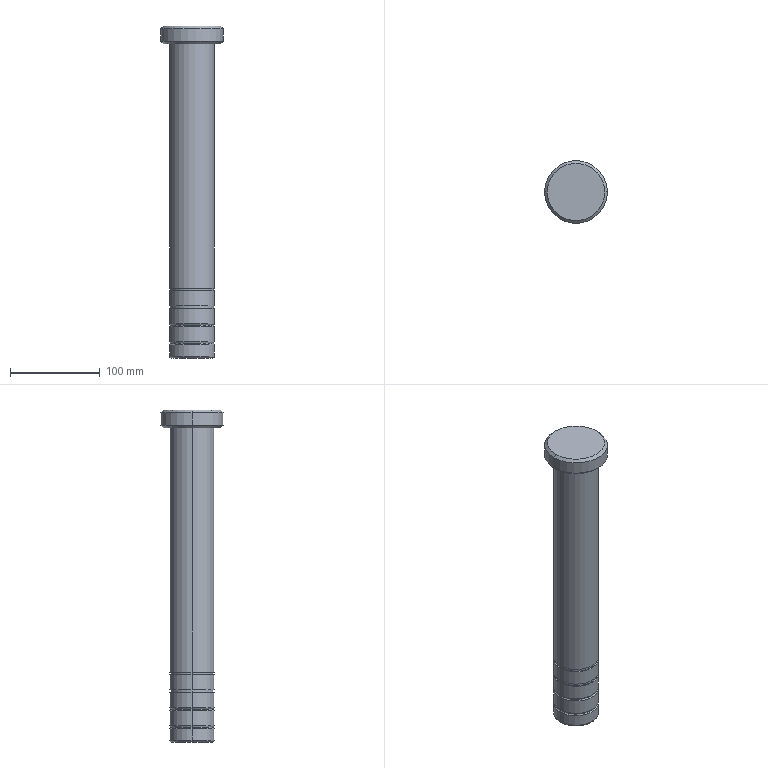Component | SolidWorks | GuidePost-1 | 1 solid | 41 faces | box 70 x 70 x 370 mm | volume 760524 mm3 | cylinder 20 | torus 10 | plane 7 | cone 4 | commonest cylinder face diameters 50 x10 48 x8 70 x2
STEP:
#1=CARTESIAN_POINT('',(-8.937,-7.677,4.921));
#2=VERTEX_POINT('',#1);
#3=CARTESIAN_POINT('',(-6.417,-7.677,4.921));
#4=VERTEX_POINT('',#3);
#5=CARTESIAN_POINT('',(-7.677,-7.677,4.921));
#6=DIRECTION('',(0.,0.,-1.));
#7=DIRECTION('',(1.,0.,0.));
#8=AXIS2_PLACEMENT_3D('',#5,#6,#7);
#9=CIRCLE('',#8,1.26);
#10=EDGE_CURVE('',#2,#4,#9,.T.);
#11=ORIENTED_EDGE('',*,*,#10,.F.);
#12=CARTESIAN_POINT('',(-9.055,-7.677,5.039));
#13=VERTEX_POINT('',#12);
#14=CARTESIAN_POINT('',(-9.055,-7.677,5.039));
#15=DIRECTION('',(-0.7071,0.,0.7071));
#16=VECTOR('',#15,39.37);
#17=LINE('',#14,#16);
#18=EDGE_CURVE('',#2,#13,#17,.T.);
#19=ORIENTED_EDGE('',*,*,#18,.T.);
#20=CARTESIAN_POINT('',(-6.299,-7.677,5.039));
#21=VERTEX_POINT('',#20);
#22=CARTESIAN_POINT('',(-7.677,-7.677,5.039));
#23=DIRECTION('',(0.,0.,1.));
#24=DIRECTION('',(1.,0.,0.));
#25=AXIS2_PLACEMENT_3D('',#22,#23,#24);
#26=CIRCLE('',#25,1.378);
#27=EDGE_CURVE('',#21,#13,#26,.T.);
#28=ORIENTED_EDGE('',*,*,#27,.F.);
#29=CARTESIAN_POINT('',(-6.299,-7.677,5.039));
#30=DIRECTION('',(0.7071,0.,0.7071));
#31=VECTOR('',#30,39.37);
#32=LINE('',#29,#31);
#33=EDGE_CURVE('',#4,#21,#32,.T.);
#34=ORIENTED_EDGE('',*,*,#33,.F.);
#35=EDGE_LOOP('',(#11,#19,#28,#34));
#36=FACE_OUTER_BOUND('',#35,.T.);
#37=CARTESIAN_POINT('',(-7.677,-7.677,5.039));
#38=DIRECTION('',(0.,0.,1.));
#39=DIRECTION('',(1.,0.,0.));
#40=AXIS2_PLACEMENT_3D('',#37,#38,#39);
#41=CONICAL_SURFACE('',#40,1.378,0.7854);
#42=ADVANCED_FACE('',(#36),#41,.T.);
#43=CARTESIAN_POINT('',(-6.417,-7.677,5.709));
#44=VERTEX_POINT('',#43);
#45=CARTESIAN_POINT('',(-8.937,-7.677,5.709));
#46=VERTEX_POINT('',#45);
#47=CARTESIAN_POINT('',(-7.677,-7.677,5.709));
#48=DIRECTION('',(0.,0.,1.));
#49=DIRECTION('',(1.,0.,0.));
#50=AXIS2_PLACEMENT_3D('',#47,#48,#49);
#51=CIRCLE('',#50,1.26);
#52=EDGE_CURVE('',#44,#46,#51,.T.);
#53=ORIENTED_EDGE('',*,*,#52,.F.);
#54=CARTESIAN_POINT('',(-6.299,-7.677,5.591));
#55=VERTEX_POINT('',#54);
#56=CARTESIAN_POINT('',(-6.417,-7.677,5.709));
#57=DIRECTION('',(0.7071,0.,-0.7071));
#58=VECTOR('',#57,39.37);
#59=LINE('',#56,#58);
#60=EDGE_CURVE('',#44,#55,#59,.T.);
#61=ORIENTED_EDGE('',*,*,#60,.T.);
#62=CARTESIAN_POINT('',(-9.055,-7.677,5.591));
#63=VERTEX_POINT('',#62);
#64=CARTESIAN_POINT('',(-7.677,-7.677,5.591));
#65=DIRECTION('',(0.,0.,-1.));
#66=DIRECTION('',(1.,0.,0.));
#67=AXIS2_PLACEMENT_3D('',#64,#65,#66);
#68=CIRCLE('',#67,1.378);
#69=EDGE_CURVE('',#63,#55,#68,.T.);
#70=ORIENTED_EDGE('',*,*,#69,.F.);
#71=CARTESIAN_POINT('',(-8.937,-7.677,5.709));
#72=DIRECTION('',(-0.7071,0.,-0.7071));
#73=VECTOR('',#72,39.37);
#74=LINE('',#71,#73);
#75=EDGE_CURVE('',#46,#63,#74,.T.);
#76=ORIENTED_EDGE('',*,*,#75,.F.);
#77=EDGE_LOOP('',(#53,#61,#70,#76));
#78=FACE_OUTER_BOUND('',#77,.T.);
#79=CARTESIAN_POINT('',(-7.677,-7.677,5.709));
#80=DIRECTION('',(0.,0.,-1.));
#81=DIRECTION('',(-1.,0.,0.));
#82=AXIS2_PLACEMENT_3D('',#79,#80,#81);
#83=CONICAL_SURFACE('',#82,1.26,0.7854);
#84=ADVANCED_FACE('',(#78),#83,.T.);
#85=CARTESIAN_POINT('',(-6.693,-7.677,-8.268));
#86=VERTEX_POINT('',#85);
#87=CARTESIAN_POINT('',(-8.661,-7.677,-8.268));
#88=VERTEX_POINT('',#87);
#89=CARTESIAN_POINT('',(-7.677,-7.677,-8.268));
#90=DIRECTION('',(0.,0.,-1.));
#91=DIRECTION('',(-1.,0.,0.));
#92=AXIS2_PLACEMENT_3D('',#89,#90,#91);
#93=CIRCLE('',#92,0.9843);
#94=EDGE_CURVE('',#86,#88,#93,.T.);
#95=ORIENTED_EDGE('',*,*,#94,.F.);
#96=CARTESIAN_POINT('',(-6.732,-7.677,-8.212));
#97=VERTEX_POINT('',#96);
#98=CARTESIAN_POINT('',(-6.673,-7.677,-8.212));
#99=DIRECTION('',(-0.,1.,0.));
#100=DIRECTION('',(-1.,0.,0.));
#101=AXIS2_PLACEMENT_3D('',#98,#99,#100);
#102=CIRCLE('',#101,0.05906);
#103=EDGE_CURVE('',#86,#97,#102,.T.);
#104=ORIENTED_EDGE('',*,*,#103,.T.);
#105=CARTESIAN_POINT('',(-8.622,-7.677,-8.212));
#106=VERTEX_POINT('',#105);
#107=CARTESIAN_POINT('',(-7.677,-7.677,-8.212));
#108=DIRECTION('',(0.,0.,1.));
#109=DIRECTION('',(-1.,0.,0.));
#110=AXIS2_PLACEMENT_3D('',#107,#108,#109);
#111=CIRCLE('',#110,0.9449);
#112=EDGE_CURVE('',#106,#97,#111,.T.);
#113=ORIENTED_EDGE('',*,*,#112,.F.);
#114=CARTESIAN_POINT('',(-8.681,-7.677,-8.212));
#115=DIRECTION('',(0.,-1.,0.));
#116=DIRECTION('',(0.,0.,-1.));
#117=AXIS2_PLACEMENT_3D('',#114,#115,#116);
#118=CIRCLE('',#117,0.05906);
#119=EDGE_CURVE('',#88,#106,#118,.T.);
#120=ORIENTED_EDGE('',*,*,#119,.F.);
#121=EDGE_LOOP('',(#95,#104,#113,#120));
#122=FACE_OUTER_BOUND('',#121,.T.);
#123=CARTESIAN_POINT('',(-7.677,-7.677,-8.212));
#124=DIRECTION('',(0.,0.,-1.));
#125=DIRECTION('',(-1.,0.,0.));
#126=AXIS2_PLACEMENT_3D('',#123,#124,#125);
#127=TOROIDAL_SURFACE('',#126,1.004,0.05906);
#128=ADVANCED_FACE('',(#122),#127,.F.);
#129=CARTESIAN_POINT('',(-6.693,-7.677,-8.15));
#130=VERTEX_POINT('',#129);
#131=CARTESIAN_POINT('',(-8.661,-7.677,-8.15));
#132=VERTEX_POINT('',#131);
#133=CARTESIAN_POINT('',(-7.677,-7.677,-8.15));
#134=DIRECTION('',(0.,0.,-1.));
#135=DIRECTION('',(-1.,0.,0.));
#136=AXIS2_PLACEMENT_3D('',#133,#134,#135);
#137=CIRCLE('',#136,0.9843);
#138=EDGE_CURVE('',#130,#132,#137,.T.);
#139=ORIENTED_EDGE('',*,*,#138,.T.);
#140=CARTESIAN_POINT('',(-8.622,-7.677,-8.205));
#141=VERTEX_POINT('',#140);
#142=CARTESIAN_POINT('',(-8.681,-7.677,-8.205));
#143=DIRECTION('',(0.,1.,0.));
#144=DIRECTION('',(-1.,0.,0.));
#145=AXIS2_PLACEMENT_3D('',#142,#143,#144);
#146=CIRCLE('',#145,0.05906);
#147=EDGE_CURVE('',#132,#141,#146,.T.);
#148=ORIENTED_EDGE('',*,*,#147,.T.);
#149=CARTESIAN_POINT('',(-6.732,-7.677,-8.205));
#150=VERTEX_POINT('',#149);
#151=CARTESIAN_POINT('',(-7.677,-7.677,-8.205));
#152=DIRECTION('',(0.,0.,-1.));
#153=DIRECTION('',(1.,0.,0.));
#154=AXIS2_PLACEMENT_3D('',#151,#152,#153);
#155=CIRCLE('',#154,0.9449);
#156=EDGE_CURVE('',#150,#141,#155,.T.);
#157=ORIENTED_EDGE('',*,*,#156,.F.);
#158=CARTESIAN_POINT('',(-6.673,-7.677,-8.205));
#159=DIRECTION('',(0.,-1.,0.));
#160=DIRECTION('',(0.,0.,-1.));
#161=AXIS2_PLACEMENT_3D('',#158,#159,#160);
#162=CIRCLE('',#161,0.05906);
#163=EDGE_CURVE('',#130,#150,#162,.T.);
#164=ORIENTED_EDGE('',*,*,#163,.F.);
#165=EDGE_LOOP('',(#139,#148,#157,#164));
#166=FACE_OUTER_BOUND('',#165,.T.);
#167=CARTESIAN_POINT('',(-7.677,-7.677,-8.205));
#168=DIRECTION('',(0.,0.,1.));
#169=DIRECTION('',(1.,0.,0.));
#170=AXIS2_PLACEMENT_3D('',#167,#168,#169);
#171=TOROIDAL_SURFACE('',#170,1.004,0.05906);
#172=ADVANCED_FACE('',(#166),#171,.F.);
#173=CARTESIAN_POINT('',(-6.693,-7.677,-7.362));
#174=VERTEX_POINT('',#173);
#175=CARTESIAN_POINT('',(-8.661,-7.677,-7.362));
#176=VERTEX_POINT('',#175);
#177=CARTESIAN_POINT('',(-7.677,-7.677,-7.362));
#178=DIRECTION('',(0.,0.,-1.));
#179=DIRECTION('',(-1.,0.,0.));
#180=AXIS2_PLACEMENT_3D('',#177,#178,#179);
#181=CIRCLE('',#180,0.9843);
#182=EDGE_CURVE('',#174,#176,#181,.T.);
#183=ORIENTED_EDGE('',*,*,#182,.T.);
#184=CARTESIAN_POINT('',(-8.622,-7.677,-7.418));
#185=VERTEX_POINT('',#184);
#186=CARTESIAN_POINT('',(-8.681,-7.677,-7.418));
#187=DIRECTION('',(0.,1.,0.));
#188=DIRECTION('',(-1.,0.,0.));
#189=AXIS2_PLACEMENT_3D('',#186,#187,#188);
#190=CIRCLE('',#189,0.05906);
#191=EDGE_CURVE('',#176,#185,#190,.T.);
#192=ORIENTED_EDGE('',*,*,#191,.T.);
#193=CARTESIAN_POINT('',(-6.732,-7.677,-7.418));
#194=VERTEX_POINT('',#193);
#195=CARTESIAN_POINT('',(-7.677,-7.677,-7.418));
#196=DIRECTION('',(0.,0.,-1.));
#197=DIRECTION('',(1.,0.,0.));
#198=AXIS2_PLACEMENT_3D('',#195,#196,#197);
#199=CIRCLE('',#198,0.9449);
#200=EDGE_CURVE('',#194,#185,#199,.T.);
#201=ORIENTED_EDGE('',*,*,#200,.F.);
#202=CARTESIAN_POINT('',(-6.673,-7.677,-7.418));
#203=DIRECTION('',(0.,-1.,0.));
#204=DIRECTION('',(0.,0.,-1.));
#205=AXIS2_PLACEMENT_3D('',#202,#203,#204);
#206=CIRCLE('',#205,0.05906);
#207=EDGE_CURVE('',#174,#194,#206,.T.);
#208=ORIENTED_EDGE('',*,*,#207,.F.);
#209=EDGE_LOOP('',(#183,#192,#201,#208));
#210=FACE_OUTER_BOUND('',#209,.T.);
#211=CARTESIAN_POINT('',(-7.677,-7.677,-7.418));
#212=DIRECTION('',(0.,0.,1.));
#213=DIRECTION('',(1.,0.,0.));
#214=AXIS2_PLACEMENT_3D('',#211,#212,#213);
#215=TOROIDAL_SURFACE('',#214,1.004,0.05906);
#216=ADVANCED_FACE('',(#210),#215,.F.);
#217=CARTESIAN_POINT('',(-6.693,-7.677,-7.48));
#218=VERTEX_POINT('',#217);
#219=CARTESIAN_POINT('',(-8.661,-7.677,-7.48));
#220=VERTEX_POINT('',#219);
#221=CARTESIAN_POINT('',(-7.677,-7.677,-7.48));
#222=DIRECTION('',(0.,0.,-1.));
#223=DIRECTION('',(-1.,0.,0.));
#224=AXIS2_PLACEMENT_3D('',#221,#222,#223);
#225=CIRCLE('',#224,0.9843);
#226=EDGE_CURVE('',#218,#220,#225,.T.);
#227=ORIENTED_EDGE('',*,*,#226,.F.);
#228=CARTESIAN_POINT('',(-6.732,-7.677,-7.425));
#229=VERTEX_POINT('',#228);
#230=CARTESIAN_POINT('',(-6.673,-7.677,-7.425));
#231=DIRECTION('',(-0.,1.,0.));
#232=DIRECTION('',(-1.,0.,0.));
#233=AXIS2_PLACEMENT_3D('',#230,#231,#232);
#234=CIRCLE('',#233,0.05906);
#235=EDGE_CURVE('',#218,#229,#234,.T.);
#236=ORIENTED_EDGE('',*,*,#235,.T.);
#237=CARTESIAN_POINT('',(-8.622,-7.677,-7.425));
#238=VERTEX_POINT('',#237);
#239=CARTESIAN_POINT('',(-7.677,-7.677,-7.425));
#240=DIRECTION('',(0.,0.,1.));
#241=DIRECTION('',(-1.,0.,0.));
#242=AXIS2_PLACEMENT_3D('',#239,#240,#241);
#243=CIRCLE('',#242,0.9449);
#244=EDGE_CURVE('',#238,#229,#243,.T.);
#245=ORIENTED_EDGE('',*,*,#244,.F.);
#246=CARTESIAN_POINT('',(-8.681,-7.677,-7.425));
#247=DIRECTION('',(0.,-1.,0.));
#248=DIRECTION('',(0.,0.,-1.));
#249=AXIS2_PLACEMENT_3D('',#246,#247,#248);
#250=CIRCLE('',#249,0.05906);
#251=EDGE_CURVE('',#220,#238,#250,.T.);
#252=ORIENTED_EDGE('',*,*,#251,.F.);
#253=EDGE_LOOP('',(#227,#236,#245,#252));
#254=FACE_OUTER_BOUND('',#253,.T.);
#255=CARTESIAN_POINT('',(-7.677,-7.677,-7.425));
#256=DIRECTION('',(0.,0.,-1.));
#257=DIRECTION('',(-1.,0.,0.));
#258=AXIS2_PLACEMENT_3D('',#255,#256,#257);
#259=TOROIDAL_SURFACE('',#258,1.004,0.05906);
#260=ADVANCED_FACE('',(#254),#259,.F.);
#261=CARTESIAN_POINT('',(-8.583,-7.677,-8.858));
#262=VERTEX_POINT('',#261);
#263=CARTESIAN_POINT('',(-6.772,-7.677,-8.858));
#264=VERTEX_POINT('',#263);
#265=CARTESIAN_POINT('',(-7.677,-7.677,-8.858));
#266=DIRECTION('',(0.,0.,-1.));
#267=DIRECTION('',(1.,0.,0.));
#268=AXIS2_PLACEMENT_3D('',#265,#266,#267);
#269=CIRCLE('',#268,0.9055);
#270=EDGE_CURVE('',#262,#264,#269,.T.);
#271=ORIENTED_EDGE('',*,*,#270,.F.);
#272=CARTESIAN_POINT('',(-8.661,-7.677,-8.78));
#273=VERTEX_POINT('',#272);
#274=CARTESIAN_POINT('',(-8.583,-7.677,-8.78));
#275=DIRECTION('',(0.,1.,0.));
#276=DIRECTION('',(-1.,0.,0.));
#277=AXIS2_PLACEMENT_3D('',#274,#275,#276);
#278=CIRCLE('',#277,0.07874);
#279=EDGE_CURVE('',#262,#273,#278,.T.);
#280=ORIENTED_EDGE('',*,*,#279,.T.);
#281=CARTESIAN_POINT('',(-6.693,-7.677,-8.78));
#282=VERTEX_POINT('',#281);
#283=CARTESIAN_POINT('',(-7.677,-7.677,-8.78));
#284=DIRECTION('',(0.,0.,1.));
#285=DIRECTION('',(1.,0.,0.));
#286=AXIS2_PLACEMENT_3D('',#283,#284,#285);
#287=CIRCLE('',#286,0.9843);
#288=EDGE_CURVE('',#282,#273,#287,.T.);
#289=ORIENTED_EDGE('',*,*,#288,.F.);
#290=CARTESIAN_POINT('',(-6.772,-7.677,-8.78));
#291=DIRECTION('',(0.,-1.,0.));
#292=DIRECTION('',(0.,0.,-1.));
#293=AXIS2_PLACEMENT_3D('',#290,#291,#292);
#294=CIRCLE('',#293,0.07874);
#295=EDGE_CURVE('',#264,#282,#294,.T.);
#296=ORIENTED_EDGE('',*,*,#295,.F.);
#297=EDGE_LOOP('',(#271,#280,#289,#296));
#298=FACE_OUTER_BOUND('',#297,.T.);
#299=CARTESIAN_POINT('',(-7.677,-7.677,-8.78));
#300=DIRECTION('',(0.,0.,1.));
#301=DIRECTION('',(1.,0.,0.));
#302=AXIS2_PLACEMENT_3D('',#299,#300,#301);
#303=TOROIDAL_SURFACE('',#302,0.9055,0.07874);
#304=ADVANCED_FACE('',(#298),#303,.T.);
#305=CARTESIAN_POINT('',(-6.693,-7.677,4.921));
#306=VERTEX_POINT('',#305);
#307=CARTESIAN_POINT('',(-8.661,-7.677,4.921));
#308=VERTEX_POINT('',#307);
#309=CARTESIAN_POINT('',(-7.677,-7.677,4.921));
#310=DIRECTION('',(0.,0.,1.));
#311=DIRECTION('',(1.,0.,0.));
#312=AXIS2_PLACEMENT_3D('',#309,#310,#311);
#313=CIRCLE('',#312,0.9843);
#314=EDGE_CURVE('',#306,#308,#313,.T.);
#315=ORIENTED_EDGE('',*,*,#314,.F.);
#316=CARTESIAN_POINT('',(-6.693,-7.677,-5.787));
#317=VERTEX_POINT('',#316);
#318=CARTESIAN_POINT('',(-6.693,-7.677,4.921));
#319=DIRECTION('',(0.,0.,-1.));
#320=VECTOR('',#319,39.37);
#321=LINE('',#318,#320);
#322=EDGE_CURVE('',#306,#317,#321,.T.);
#323=ORIENTED_EDGE('',*,*,#322,.T.);
#324=CARTESIAN_POINT('',(-8.661,-7.677,-5.787));
#325=VERTEX_POINT('',#324);
#326=CARTESIAN_POINT('',(-7.677,-7.677,-5.787));
#327=DIRECTION('',(0.,0.,-1.));
#328=DIRECTION('',(-1.,0.,0.));
#329=AXIS2_PLACEMENT_3D('',#326,#327,#328);
#330=CIRCLE('',#329,0.9843);
#331=EDGE_CURVE('',#325,#317,#330,.T.);
#332=ORIENTED_EDGE('',*,*,#331,.F.);
#333=CARTESIAN_POINT('',(-8.661,-7.677,4.921));
#334=DIRECTION('',(0.,0.,-1.));
#335=VECTOR('',#334,39.37);
#336=LINE('',#333,#335);
#337=EDGE_CURVE('',#308,#325,#336,.T.);
#338=ORIENTED_EDGE('',*,*,#337,.F.);
#339=EDGE_LOOP('',(#315,#323,#332,#338));
#340=FACE_OUTER_BOUND('',#339,.T.);
#341=CARTESIAN_POINT('',(-7.677,-7.677,4.921));
#342=DIRECTION('',(0.,0.,-1.));
#343=DIRECTION('',(-1.,0.,0.));
#344=AXIS2_PLACEMENT_3D('',#341,#342,#343);
#345=CYLINDRICAL_SURFACE('',#344,0.9843);
#346=ADVANCED_FACE('',(#340),#345,.T.);
#347=ORIENTED_EDGE('',*,*,#69,.T.);
#348=CARTESIAN_POINT('',(-6.299,-7.677,5.709));
#349=DIRECTION('',(0.,0.,-1.));
#350=VECTOR('',#349,39.37);
#351=LINE('',#348,#350);
#352=EDGE_CURVE('',#55,#21,#351,.T.);
#353=ORIENTED_EDGE('',*,*,#352,.T.);
#354=ORIENTED_EDGE('',*,*,#27,.T.);
#355=CARTESIAN_POINT('',(-9.055,-7.677,5.709));
#356=DIRECTION('',(0.,0.,-1.));
#357=VECTOR('',#356,39.37);
#358=LINE('',#355,#357);
#359=EDGE_CURVE('',#63,#13,#358,.T.);
#360=ORIENTED_EDGE('',*,*,#359,.F.);
#361=EDGE_LOOP('',(#347,#353,#354,#360));
#362=FACE_OUTER_BOUND('',#361,.T.);
#363=CARTESIAN_POINT('',(-7.677,-7.677,5.709));
#364=DIRECTION('',(0.,0.,-1.));
#365=DIRECTION('',(-1.,0.,0.));
#366=AXIS2_PLACEMENT_3D('',#363,#364,#365);
#367=CYLINDRICAL_SURFACE('',#366,1.378);
#368=ADVANCED_FACE('',(#362),#367,.T.);
#369=CARTESIAN_POINT('',(-8.622,-7.677,-5.787));
#370=VERTEX_POINT('',#369);
#371=CARTESIAN_POINT('',(-6.732,-7.677,-5.787));
#372=VERTEX_POINT('',#371);
#373=CARTESIAN_POINT('',(-7.677,-7.677,-5.787));
#374=DIRECTION('',(0.,0.,-1.));
#375=DIRECTION('',(-1.,0.,0.));
#376=AXIS2_PLACEMENT_3D('',#373,#374,#375);
#377=CIRCLE('',#376,0.9449);
#378=EDGE_CURVE('',#370,#372,#377,.T.);
#379=ORIENTED_EDGE('',*,*,#378,.T.);
#380=CARTESIAN_POINT('',(-6.732,-7.677,-5.906));
#381=VERTEX_POINT('',#380);
#382=CARTESIAN_POINT('',(-6.732,-7.677,-5.787));
#383=DIRECTION('',(0.,0.,-1.));
#384=VECTOR('',#383,39.37);
#385=LINE('',#382,#384);
#386=EDGE_CURVE('',#372,#381,#385,.T.);
#387=ORIENTED_EDGE('',*,*,#386,.T.);
#388=CARTESIAN_POINT('',(-8.622,-7.677,-5.906));
#389=VERTEX_POINT('',#388);
#390=CARTESIAN_POINT('',(-7.677,-7.677,-5.906));
#391=DIRECTION('',(0.,0.,-1.));
#392=DIRECTION('',(-1.,0.,0.));
#393=AXIS2_PLACEMENT_3D('',#390,#391,#392);
#394=CIRCLE('',#393,0.9449);
#395=EDGE_CURVE('',#389,#381,#394,.T.);
#396=ORIENTED_EDGE('',*,*,#395,.F.);
#397=CARTESIAN_POINT('',(-8.622,-7.677,-5.787));
#398=DIRECTION('',(0.,0.,-1.));
#399=VECTOR('',#398,39.37);
#400=LINE('',#397,#399);
#401=EDGE_CURVE('',#370,#389,#400,.T.);
#402=ORIENTED_EDGE('',*,*,#401,.F.);
#403=EDGE_LOOP('',(#379,#387,#396,#402));
#404=FACE_OUTER_BOUND('',#403,.T.);
#405=CARTESIAN_POINT('',(-7.677,-7.677,-5.787));
#406=DIRECTION('',(0.,0.,-1.));
#407=DIRECTION('',(-1.,0.,0.));
#408=AXIS2_PLACEMENT_3D('',#405,#406,#407);
#409=CYLINDRICAL_SURFACE('',#408,0.9449);
#410=ADVANCED_FACE('',(#404),#409,.T.);
#411=CARTESIAN_POINT('',(-8.661,-7.677,-5.906));
#412=VERTEX_POINT('',#411);
#413=CARTESIAN_POINT('',(-6.693,-7.677,-5.906));
#414=VERTEX_POINT('',#413);
#415=CARTESIAN_POINT('',(-7.677,-7.677,-5.906));
#416=DIRECTION('',(0.,0.,-1.));
#417=DIRECTION('',(-1.,0.,0.));
#418=AXIS2_PLACEMENT_3D('',#415,#416,#417);
#419=CIRCLE('',#418,0.9843);
#420=EDGE_CURVE('',#412,#414,#419,.T.);
#421=ORIENTED_EDGE('',*,*,#420,.T.);
#422=CARTESIAN_POINT('',(-6.693,-7.677,-6.575));
#423=VERTEX_POINT('',#422);
#424=CARTESIAN_POINT('',(-6.693,-7.677,4.921));
#425=DIRECTION('',(0.,0.,-1.));
#426=VECTOR('',#425,39.37);
#427=LINE('',#424,#426);
#428=EDGE_CURVE('',#414,#423,#427,.T.);
#429=ORIENTED_EDGE('',*,*,#428,.T.);
#430=CARTESIAN_POINT('',(-8.661,-7.677,-6.575));
#431=VERTEX_POINT('',#430);
#432=CARTESIAN_POINT('',(-7.677,-7.677,-6.575));
#433=DIRECTION('',(0.,0.,-1.));
#434=DIRECTION('',(-1.,0.,0.));
#435=AXIS2_PLACEMENT_3D('',#432,#433,#434);
#436=CIRCLE('',#435,0.9843);
#437=EDGE_CURVE('',#431,#423,#436,.T.);
#438=ORIENTED_EDGE('',*,*,#437,.F.);
#439=CARTESIAN_POINT('',(-8.661,-7.677,4.921));
#440=DIRECTION('',(0.,0.,-1.));
#441=VECTOR('',#440,39.37);
#442=LINE('',#439,#441);
#443=EDGE_CURVE('',#412,#431,#442,.T.);
#444=ORIENTED_EDGE('',*,*,#443,.F.);
#445=EDGE_LOOP('',(#421,#429,#438,#444));
#446=FACE_OUTER_BOUND('',#445,.T.);
#447=CARTESIAN_POINT('',(-7.677,-7.677,4.921));
#448=DIRECTION('',(0.,0.,-1.));
#449=DIRECTION('',(-1.,0.,0.));
#450=AXIS2_PLACEMENT_3D('',#447,#448,#449);
#451=CYLINDRICAL_SURFACE('',#450,0.9843);
#452=ADVANCED_FACE('',(#446),#451,.T.);
#453=CARTESIAN_POINT('',(-8.622,-7.677,-6.575));
#454=VERTEX_POINT('',#453);
#455=CARTESIAN_POINT('',(-6.732,-7.677,-6.575));
#456=VERTEX_POINT('',#455);
#457=CARTESIAN_POINT('',(-7.677,-7.677,-6.575));
#458=DIRECTION('',(0.,0.,-1.));
#459=DIRECTION('',(-1.,0.,0.));
#460=AXIS2_PLACEMENT_3D('',#457,#458,#459);
#461=CIRCLE('',#460,0.9449);
#462=EDGE_CURVE('',#454,#456,#461,.T.);
#463=ORIENTED_EDGE('',*,*,#462,.T.);
#464=CARTESIAN_POINT('',(-6.732,-7.677,-6.693));
#465=VERTEX_POINT('',#464);
#466=CARTESIAN_POINT('',(-6.732,-7.677,-6.575));
#467=DIRECTION('',(0.,0.,-1.));
#468=VECTOR('',#467,39.37);
#469=LINE('',#466,#468);
#470=EDGE_CURVE('',#456,#465,#469,.T.);
#471=ORIENTED_EDGE('',*,*,#470,.T.);
#472=CARTESIAN_POINT('',(-8.622,-7.677,-6.693));
#473=VERTEX_POINT('',#472);
#474=CARTESIAN_POINT('',(-7.677,-7.677,-6.693));
#475=DIRECTION('',(0.,0.,-1.));
#476=DIRECTION('',(-1.,0.,0.));
#477=AXIS2_PLACEMENT_3D('',#474,#475,#476);
#478=CIRCLE('',#477,0.9449);
#479=EDGE_CURVE('',#473,#465,#478,.T.);
#480=ORIENTED_EDGE('',*,*,#479,.F.);
#481=CARTESIAN_POINT('',(-8.622,-7.677,-6.575));
#482=DIRECTION('',(0.,0.,-1.));
#483=VECTOR('',#482,39.37);
#484=LINE('',#481,#483);
#485=EDGE_CURVE('',#454,#473,#484,.T.);
#486=ORIENTED_EDGE('',*,*,#485,.F.);
#487=EDGE_LOOP('',(#463,#471,#480,#486));
#488=FACE_OUTER_BOUND('',#487,.T.);
#489=CARTESIAN_POINT('',(-7.677,-7.677,-6.575));
#490=DIRECTION('',(0.,0.,-1.));
#491=DIRECTION('',(-1.,0.,0.));
#492=AXIS2_PLACEMENT_3D('',#489,#490,#491);
#493=CYLINDRICAL_SURFACE('',#492,0.9449);
#494=ADVANCED_FACE('',(#488),#493,.T.);
#495=CARTESIAN_POINT('',(-8.661,-7.677,-6.693));
#496=VERTEX_POINT('',#495);
#497=CARTESIAN_POINT('',(-6.693,-7.677,-6.693));
#498=VERTEX_POINT('',#497);
#499=CARTESIAN_POINT('',(-7.677,-7.677,-6.693));
#500=DIRECTION('',(0.,0.,-1.));
#501=DIRECTION('',(-1.,0.,0.));
#502=AXIS2_PLACEMENT_3D('',#499,#500,#501);
#503=CIRCLE('',#502,0.9843);
#504=EDGE_CURVE('',#496,#498,#503,.T.);
#505=ORIENTED_EDGE('',*,*,#504,.T.);
#506=CARTESIAN_POINT('',(-6.693,-7.677,4.921));
#507=DIRECTION('',(0.,0.,-1.));
#508=VECTOR('',#507,39.37);
#509=LINE('',#506,#508);
#510=EDGE_CURVE('',#498,#174,#509,.T.);
#511=ORIENTED_EDGE('',*,*,#510,.T.);
#512=CARTESIAN_POINT('',(-7.677,-7.677,-7.362));
#513=DIRECTION('',(0.,0.,-1.));
#514=DIRECTION('',(-1.,0.,0.));
#515=AXIS2_PLACEMENT_3D('',#512,#513,#514);
#516=CIRCLE('',#515,0.9843);
#517=EDGE_CURVE('',#176,#174,#516,.T.);
#518=ORIENTED_EDGE('',*,*,#517,.F.);
#519=CARTESIAN_POINT('',(-8.661,-7.677,4.921));
#520=DIRECTION('',(0.,0.,-1.));
#521=VECTOR('',#520,39.37);
#522=LINE('',#519,#521);
#523=EDGE_CURVE('',#496,#176,#522,.T.);
#524=ORIENTED_EDGE('',*,*,#523,.F.);
#525=EDGE_LOOP('',(#505,#511,#518,#524));
#526=FACE_OUTER_BOUND('',#525,.T.);
#527=CARTESIAN_POINT('',(-7.677,-7.677,4.921));
#528=DIRECTION('',(0.,0.,-1.));
#529=DIRECTION('',(-1.,0.,0.));
#530=AXIS2_PLACEMENT_3D('',#527,#528,#529);
#531=CYLINDRICAL_SURFACE('',#530,0.9843);
#532=ADVANCED_FACE('',(#526),#531,.T.);
#533=CARTESIAN_POINT('',(-7.677,-7.677,-7.418));
#534=DIRECTION('',(0.,0.,-1.));
#535=DIRECTION('',(1.,0.,0.));
#536=AXIS2_PLACEMENT_3D('',#533,#534,#535);
#537=CIRCLE('',#536,0.9449);
#538=EDGE_CURVE('',#185,#194,#537,.T.);
#539=ORIENTED_EDGE('',*,*,#538,.T.);
#540=CARTESIAN_POINT('',(-6.732,-7.677,-7.362));
#541=DIRECTION('',(0.,0.,-1.));
#542=VECTOR('',#541,39.37);
#543=LINE('',#540,#542);
#544=EDGE_CURVE('',#194,#229,#543,.T.);
#545=ORIENTED_EDGE('',*,*,#544,.T.);
#546=CARTESIAN_POINT('',(-7.677,-7.677,-7.425));
#547=DIRECTION('',(0.,0.,1.));
#548=DIRECTION('',(-1.,0.,0.));
#549=AXIS2_PLACEMENT_3D('',#546,#547,#548);
#550=CIRCLE('',#549,0.9449);
#551=EDGE_CURVE('',#229,#238,#550,.T.);
#552=ORIENTED_EDGE('',*,*,#551,.T.);
#553=CARTESIAN_POINT('',(-8.622,-7.677,-7.362));
#554=DIRECTION('',(0.,0.,-1.));
#555=VECTOR('',#554,39.37);
#556=LINE('',#553,#555);
#557=EDGE_CURVE('',#185,#238,#556,.T.);
#558=ORIENTED_EDGE('',*,*,#557,.F.);
#559=EDGE_LOOP('',(#539,#545,#552,#558));
#560=FACE_OUTER_BOUND('',#559,.T.);
#561=CARTESIAN_POINT('',(-7.677,-7.677,-7.362));
#562=DIRECTION('',(0.,0.,-1.));
#563=DIRECTION('',(-1.,0.,0.));
#564=AXIS2_PLACEMENT_3D('',#561,#562,#563);
#565=CYLINDRICAL_SURFACE('',#564,0.9449);
#566=ADVANCED_FACE('',(#560),#565,.T.);
#567=CARTESIAN_POINT('',(-7.677,-7.677,-8.268));
#568=DIRECTION('',(0.,0.,-1.));
#569=DIRECTION('',(-1.,0.,0.));
#570=AXIS2_PLACEMENT_3D('',#567,#568,#569);
#571=CIRCLE('',#570,0.9843);
#572=EDGE_CURVE('',#88,#86,#571,.T.);
#573=ORIENTED_EDGE('',*,*,#572,.T.);
#574=CARTESIAN_POINT('',(-6.693,-7.677,4.921));
#575=DIRECTION('',(0.,0.,-1.));
#576=VECTOR('',#575,39.37);
#577=LINE('',#574,#576);
#578=EDGE_CURVE('',#86,#282,#577,.T.);
#579=ORIENTED_EDGE('',*,*,#578,.T.);
#580=ORIENTED_EDGE('',*,*,#288,.T.);
#581=CARTESIAN_POINT('',(-8.661,-7.677,4.921));
#582=DIRECTION('',(0.,0.,-1.));
#583=VECTOR('',#582,39.37);
#584=LINE('',#581,#583);
#585=EDGE_CURVE('',#88,#273,#584,.T.);
#586=ORIENTED_EDGE('',*,*,#585,.F.);
#587=EDGE_LOOP('',(#573,#579,#580,#586));
#588=FACE_OUTER_BOUND('',#587,.T.);
#589=CARTESIAN_POINT('',(-7.677,-7.677,4.921));
#590=DIRECTION('',(0.,0.,-1.));
#591=DIRECTION('',(-1.,0.,0.));
#592=AXIS2_PLACEMENT_3D('',#589,#590,#591);
#593=CYLINDRICAL_SURFACE('',#592,0.9843);
#594=ADVANCED_FACE('',(#588),#593,.T.);
#595=CARTESIAN_POINT('',(-7.677,-7.677,-8.205));
#596=DIRECTION('',(0.,0.,-1.));
#597=DIRECTION('',(1.,0.,0.));
#598=AXIS2_PLACEMENT_3D('',#595,#596,#597);
#599=CIRCLE('',#598,0.9449);
#600=EDGE_CURVE('',#141,#150,#599,.T.);
#601=ORIENTED_EDGE('',*,*,#600,.T.);
#602=CARTESIAN_POINT('',(-6.732,-7.677,-8.15));
#603=DIRECTION('',(0.,0.,-1.));
#604=VECTOR('',#603,39.37);
#605=LINE('',#602,#604);
#606=EDGE_CURVE('',#150,#97,#605,.T.);
#607=ORIENTED_EDGE('',*,*,#606,.T.);
#608=CARTESIAN_POINT('',(-7.677,-7.677,-8.212));
#609=DIRECTION('',(0.,0.,1.));
#610=DIRECTION('',(-1.,0.,0.));
#611=AXIS2_PLACEMENT_3D('',#608,#609,#610);
#612=CIRCLE('',#611,0.9449);
#613=EDGE_CURVE('',#97,#106,#612,.T.);
#614=ORIENTED_EDGE('',*,*,#613,.T.);
#615=CARTESIAN_POINT('',(-8.622,-7.677,-8.15));
#616=DIRECTION('',(0.,0.,-1.));
#617=VECTOR('',#616,39.37);
#618=LINE('',#615,#617);
#619=EDGE_CURVE('',#141,#106,#618,.T.);
#620=ORIENTED_EDGE('',*,*,#619,.F.);
#621=EDGE_LOOP('',(#601,#607,#614,#620));
#622=FACE_OUTER_BOUND('',#621,.T.);
#623=CARTESIAN_POINT('',(-7.677,-7.677,-8.15));
#624=DIRECTION('',(0.,0.,-1.));
#625=DIRECTION('',(-1.,0.,0.));
#626=AXIS2_PLACEMENT_3D('',#623,#624,#625);
#627=CYLINDRICAL_SURFACE('',#626,0.9449);
#628=ADVANCED_FACE('',(#622),#627,.T.);
#629=CARTESIAN_POINT('',(-7.677,-7.677,-7.48));
#630=DIRECTION('',(0.,0.,-1.));
#631=DIRECTION('',(-1.,0.,0.));
#632=AXIS2_PLACEMENT_3D('',#629,#630,#631);
#633=CIRCLE('',#632,0.9843);
#634=EDGE_CURVE('',#220,#218,#633,.T.);
#635=ORIENTED_EDGE('',*,*,#634,.T.);
#636=CARTESIAN_POINT('',(-6.693,-7.677,4.921));
#637=DIRECTION('',(0.,0.,-1.));
#638=VECTOR('',#637,39.37);
#639=LINE('',#636,#638);
#640=EDGE_CURVE('',#218,#130,#639,.T.);
#641=ORIENTED_EDGE('',*,*,#640,.T.);
#642=CARTESIAN_POINT('',(-7.677,-7.677,-8.15));
#643=DIRECTION('',(0.,0.,-1.));
#644=DIRECTION('',(-1.,0.,0.));
#645=AXIS2_PLACEMENT_3D('',#642,#643,#644);
#646=CIRCLE('',#645,0.9843);
#647=EDGE_CURVE('',#132,#130,#646,.T.);
#648=ORIENTED_EDGE('',*,*,#647,.F.);
#649=CARTESIAN_POINT('',(-8.661,-7.677,4.921));
#650=DIRECTION('',(0.,0.,-1.));
#651=VECTOR('',#650,39.37);
#652=LINE('',#649,#651);
#653=EDGE_CURVE('',#220,#132,#652,.T.);
#654=ORIENTED_EDGE('',*,*,#653,.F.);
#655=EDGE_LOOP('',(#635,#641,#648,#654));
#656=FACE_OUTER_BOUND('',#655,.T.);
#657=CARTESIAN_POINT('',(-7.677,-7.677,4.921));
#658=DIRECTION('',(0.,0.,-1.));
#659=DIRECTION('',(-1.,0.,0.));
#660=AXIS2_PLACEMENT_3D('',#657,#658,#659);
#661=CYLINDRICAL_SURFACE('',#660,0.9843);
#662=ADVANCED_FACE('',(#656),#661,.T.);
#663=ORIENTED_EDGE('',*,*,#640,.F.);
#664=ORIENTED_EDGE('',*,*,#226,.T.);
#665=ORIENTED_EDGE('',*,*,#653,.T.);
#666=ORIENTED_EDGE('',*,*,#138,.F.);
#667=EDGE_LOOP('',(#663,#664,#665,#666));
#668=FACE_OUTER_BOUND('',#667,.T.);
#669=CARTESIAN_POINT('',(-7.677,-7.677,4.921));
#670=DIRECTION('',(0.,0.,-1.));
#671=DIRECTION('',(-1.,0.,0.));
#672=AXIS2_PLACEMENT_3D('',#669,#670,#671);
#673=CYLINDRICAL_SURFACE('',#672,0.9843);
#674=ADVANCED_FACE('',(#668),#673,.T.);
#675=ORIENTED_EDGE('',*,*,#606,.F.);
#676=ORIENTED_EDGE('',*,*,#156,.T.);
#677=ORIENTED_EDGE('',*,*,#619,.T.);
#678=ORIENTED_EDGE('',*,*,#112,.T.);
#679=EDGE_LOOP('',(#675,#676,#677,#678));
#680=FACE_OUTER_BOUND('',#679,.T.);
#681=CARTESIAN_POINT('',(-7.677,-7.677,-8.15));
#682=DIRECTION('',(0.,0.,-1.));
#683=DIRECTION('',(-1.,0.,0.));
#684=AXIS2_PLACEMENT_3D('',#681,#682,#683);
#685=CYLINDRICAL_SURFACE('',#684,0.9449);
#686=ADVANCED_FACE('',(#680),#685,.T.);
#687=CARTESIAN_POINT('',(-7.677,-7.677,-8.858));
#688=DIRECTION('',(0.,0.,-1.));
#689=DIRECTION('',(1.,0.,0.));
#690=AXIS2_PLACEMENT_3D('',#687,#688,#689);
#691=CIRCLE('',#690,0.9055);
#692=EDGE_CURVE('',#264,#262,#691,.T.);
#693=ORIENTED_EDGE('',*,*,#692,.T.);
#694=ORIENTED_EDGE('',*,*,#270,.T.);
#695=EDGE_LOOP('',(#693,#694));
#696=FACE_OUTER_BOUND('',#695,.T.);
#697=CARTESIAN_POINT('',(-7.677,-7.677,-8.858));
#698=DIRECTION('',(0.,0.,1.));
#699=DIRECTION('',(1.,0.,0.));
#700=AXIS2_PLACEMENT_3D('',#697,#698,#699);
#701=PLANE('',#700);
#702=ADVANCED_FACE('',(#696),#701,.F.);
#703=ORIENTED_EDGE('',*,*,#578,.F.);
#704=ORIENTED_EDGE('',*,*,#94,.T.);
#705=ORIENTED_EDGE('',*,*,#585,.T.);
#706=CARTESIAN_POINT('',(-7.677,-7.677,-8.78));
#707=DIRECTION('',(0.,0.,1.));
#708=DIRECTION('',(1.,0.,0.));
#709=AXIS2_PLACEMENT_3D('',#706,#707,#708);
#710=CIRCLE('',#709,0.9843);
#711=EDGE_CURVE('',#273,#282,#710,.T.);
#712=ORIENTED_EDGE('',*,*,#711,.T.);
#713=EDGE_LOOP('',(#703,#704,#705,#712));
#714=FACE_OUTER_BOUND('',#713,.T.);
#715=CARTESIAN_POINT('',(-7.677,-7.677,4.921));
#716=DIRECTION('',(0.,0.,-1.));
#717=DIRECTION('',(-1.,0.,0.));
#718=AXIS2_PLACEMENT_3D('',#715,#716,#717);
#719=CYLINDRICAL_SURFACE('',#718,0.9843);
#720=ADVANCED_FACE('',(#714),#719,.T.);
#721=ORIENTED_EDGE('',*,*,#544,.F.);
#722=ORIENTED_EDGE('',*,*,#200,.T.);
#723=ORIENTED_EDGE('',*,*,#557,.T.);
#724=ORIENTED_EDGE('',*,*,#244,.T.);
#725=EDGE_LOOP('',(#721,#722,#723,#724));
#726=FACE_OUTER_BOUND('',#725,.T.);
#727=CARTESIAN_POINT('',(-7.677,-7.677,-7.362));
#728=DIRECTION('',(0.,0.,-1.));
#729=DIRECTION('',(-1.,0.,0.));
#730=AXIS2_PLACEMENT_3D('',#727,#728,#729);
#731=CYLINDRICAL_SURFACE('',#730,0.9449);
#732=ADVANCED_FACE('',(#726),#731,.T.);
#733=ORIENTED_EDGE('',*,*,#510,.F.);
#734=CARTESIAN_POINT('',(-7.677,-7.677,-6.693));
#735=DIRECTION('',(0.,0.,-1.));
#736=DIRECTION('',(-1.,0.,0.));
#737=AXIS2_PLACEMENT_3D('',#734,#735,#736);
#738=CIRCLE('',#737,0.9843);
#739=EDGE_CURVE('',#498,#496,#738,.T.);
#740=ORIENTED_EDGE('',*,*,#739,.T.);
#741=ORIENTED_EDGE('',*,*,#523,.T.);
#742=ORIENTED_EDGE('',*,*,#182,.F.);
#743=EDGE_LOOP('',(#733,#740,#741,#742));
#744=FACE_OUTER_BOUND('',#743,.T.);
#745=CARTESIAN_POINT('',(-7.677,-7.677,4.921));
#746=DIRECTION('',(0.,0.,-1.));
#747=DIRECTION('',(-1.,0.,0.));
#748=AXIS2_PLACEMENT_3D('',#745,#746,#747);
#749=CYLINDRICAL_SURFACE('',#748,0.9843);
#750=ADVANCED_FACE('',(#744),#749,.T.);
#751=ORIENTED_EDGE('',*,*,#462,.F.);
#752=CARTESIAN_POINT('',(-7.677,-7.677,-6.575));
#753=DIRECTION('',(0.,0.,-1.));
#754=DIRECTION('',(-1.,0.,0.));
#755=AXIS2_PLACEMENT_3D('',#752,#753,#754);
#756=CIRCLE('',#755,0.9449);
#757=EDGE_CURVE('',#456,#454,#756,.T.);
#758=ORIENTED_EDGE('',*,*,#757,.F.);
#759=EDGE_LOOP('',(#751,#758));
#760=FACE_BOUND('',#759,.T.);
#761=ORIENTED_EDGE('',*,*,#437,.T.);
#762=CARTESIAN_POINT('',(-7.677,-7.677,-6.575));
#763=DIRECTION('',(0.,0.,-1.));
#764=DIRECTION('',(-1.,0.,0.));
#765=AXIS2_PLACEMENT_3D('',#762,#763,#764);
#766=CIRCLE('',#765,0.9843);
#767=EDGE_CURVE('',#423,#431,#766,.T.);
#768=ORIENTED_EDGE('',*,*,#767,.T.);
#769=EDGE_LOOP('',(#761,#768));
#770=FACE_OUTER_BOUND('',#769,.T.);
#771=CARTESIAN_POINT('',(-7.677,-7.677,-6.575));
#772=DIRECTION('',(0.,0.,-1.));
#773=DIRECTION('',(-1.,0.,0.));
#774=AXIS2_PLACEMENT_3D('',#771,#772,#773);
#775=PLANE('',#774);
#776=ADVANCED_FACE('',(#760,#770),#775,.T.);
#777=ORIENTED_EDGE('',*,*,#479,.T.);
#778=CARTESIAN_POINT('',(-7.677,-7.677,-6.693));
#779=DIRECTION('',(0.,0.,-1.));
#780=DIRECTION('',(-1.,0.,0.));
#781=AXIS2_PLACEMENT_3D('',#778,#779,#780);
#782=CIRCLE('',#781,0.9449);
#783=EDGE_CURVE('',#465,#473,#782,.T.);
#784=ORIENTED_EDGE('',*,*,#783,.T.);
#785=EDGE_LOOP('',(#777,#784));
#786=FACE_BOUND('',#785,.T.);
#787=ORIENTED_EDGE('',*,*,#504,.F.);
#788=ORIENTED_EDGE('',*,*,#739,.F.);
#789=EDGE_LOOP('',(#787,#788));
#790=FACE_OUTER_BOUND('',#789,.T.);
#791=CARTESIAN_POINT('',(-7.677,-7.677,-6.693));
#792=DIRECTION('',(0.,0.,-1.));
#793=DIRECTION('',(-1.,0.,0.));
#794=AXIS2_PLACEMENT_3D('',#791,#792,#793);
#795=PLANE('',#794);
#796=ADVANCED_FACE('',(#786,#790),#795,.F.);
#797=ORIENTED_EDGE('',*,*,#470,.F.);
#798=ORIENTED_EDGE('',*,*,#757,.T.);
#799=ORIENTED_EDGE('',*,*,#485,.T.);
#800=ORIENTED_EDGE('',*,*,#783,.F.);
#801=EDGE_LOOP('',(#797,#798,#799,#800));
#802=FACE_OUTER_BOUND('',#801,.T.);
#803=CARTESIAN_POINT('',(-7.677,-7.677,-6.575));
#804=DIRECTION('',(0.,0.,-1.));
#805=DIRECTION('',(-1.,0.,0.));
#806=AXIS2_PLACEMENT_3D('',#803,#804,#805);
#807=CYLINDRICAL_SURFACE('',#806,0.9449);
#808=ADVANCED_FACE('',(#802),#807,.T.);
#809=ORIENTED_EDGE('',*,*,#428,.F.);
#810=CARTESIAN_POINT('',(-7.677,-7.677,-5.906));
#811=DIRECTION('',(0.,0.,-1.));
#812=DIRECTION('',(-1.,0.,0.));
#813=AXIS2_PLACEMENT_3D('',#810,#811,#812);
#814=CIRCLE('',#813,0.9843);
#815=EDGE_CURVE('',#414,#412,#814,.T.);
#816=ORIENTED_EDGE('',*,*,#815,.T.);
#817=ORIENTED_EDGE('',*,*,#443,.T.);
#818=ORIENTED_EDGE('',*,*,#767,.F.);
#819=EDGE_LOOP('',(#809,#816,#817,#818));
#820=FACE_OUTER_BOUND('',#819,.T.);
#821=CARTESIAN_POINT('',(-7.677,-7.677,4.921));
#822=DIRECTION('',(0.,0.,-1.));
#823=DIRECTION('',(-1.,0.,0.));
#824=AXIS2_PLACEMENT_3D('',#821,#822,#823);
#825=CYLINDRICAL_SURFACE('',#824,0.9843);
#826=ADVANCED_FACE('',(#820),#825,.T.);
#827=ORIENTED_EDGE('',*,*,#378,.F.);
#828=CARTESIAN_POINT('',(-7.677,-7.677,-5.787));
#829=DIRECTION('',(0.,0.,-1.));
#830=DIRECTION('',(-1.,0.,0.));
#831=AXIS2_PLACEMENT_3D('',#828,#829,#830);
#832=CIRCLE('',#831,0.9449);
#833=EDGE_CURVE('',#372,#370,#832,.T.);
#834=ORIENTED_EDGE('',*,*,#833,.F.);
#835=EDGE_LOOP('',(#827,#834));
#836=FACE_BOUND('',#835,.T.);
#837=ORIENTED_EDGE('',*,*,#331,.T.);
#838=CARTESIAN_POINT('',(-7.677,-7.677,-5.787));
#839=DIRECTION('',(0.,0.,-1.));
#840=DIRECTION('',(-1.,0.,0.));
#841=AXIS2_PLACEMENT_3D('',#838,#839,#840);
#842=CIRCLE('',#841,0.9843);
#843=EDGE_CURVE('',#317,#325,#842,.T.);
#844=ORIENTED_EDGE('',*,*,#843,.T.);
#845=EDGE_LOOP('',(#837,#844));
#846=FACE_OUTER_BOUND('',#845,.T.);
#847=CARTESIAN_POINT('',(-7.677,-7.677,-5.787));
#848=DIRECTION('',(0.,0.,-1.));
#849=DIRECTION('',(-1.,0.,0.));
#850=AXIS2_PLACEMENT_3D('',#847,#848,#849);
#851=PLANE('',#850);
#852=ADVANCED_FACE('',(#836,#846),#851,.T.);
#853=ORIENTED_EDGE('',*,*,#395,.T.);
#854=CARTESIAN_POINT('',(-7.677,-7.677,-5.906));
#855=DIRECTION('',(0.,0.,-1.));
#856=DIRECTION('',(-1.,0.,0.));
#857=AXIS2_PLACEMENT_3D('',#854,#855,#856);
#858=CIRCLE('',#857,0.9449);
#859=EDGE_CURVE('',#381,#389,#858,.T.);
#860=ORIENTED_EDGE('',*,*,#859,.T.);
#861=EDGE_LOOP('',(#853,#860));
#862=FACE_BOUND('',#861,.T.);
#863=ORIENTED_EDGE('',*,*,#420,.F.);
#864=ORIENTED_EDGE('',*,*,#815,.F.);
#865=EDGE_LOOP('',(#863,#864));
#866=FACE_OUTER_BOUND('',#865,.T.);
#867=CARTESIAN_POINT('',(-7.677,-7.677,-5.906));
#868=DIRECTION('',(0.,0.,-1.));
#869=DIRECTION('',(-1.,0.,0.));
#870=AXIS2_PLACEMENT_3D('',#867,#868,#869);
#871=PLANE('',#870);
#872=ADVANCED_FACE('',(#862,#866),#871,.F.);
#873=ORIENTED_EDGE('',*,*,#386,.F.);
#874=ORIENTED_EDGE('',*,*,#833,.T.);
#875=ORIENTED_EDGE('',*,*,#401,.T.);
#876=ORIENTED_EDGE('',*,*,#859,.F.);
#877=EDGE_LOOP('',(#873,#874,#875,#876));
#878=FACE_OUTER_BOUND('',#877,.T.);
#879=CARTESIAN_POINT('',(-7.677,-7.677,-5.787));
#880=DIRECTION('',(0.,0.,-1.));
#881=DIRECTION('',(-1.,0.,0.));
#882=AXIS2_PLACEMENT_3D('',#879,#880,#881);
#883=CYLINDRICAL_SURFACE('',#882,0.9449);
#884=ADVANCED_FACE('',(#878),#883,.T.);
#885=CARTESIAN_POINT('',(-7.677,-7.677,5.709));
#886=DIRECTION('',(0.,0.,1.));
#887=DIRECTION('',(1.,0.,0.));
#888=AXIS2_PLACEMENT_3D('',#885,#886,#887);
#889=CIRCLE('',#888,1.26);
#890=EDGE_CURVE('',#46,#44,#889,.T.);
#891=ORIENTED_EDGE('',*,*,#890,.T.);
#892=ORIENTED_EDGE('',*,*,#52,.T.);
#893=EDGE_LOOP('',(#891,#892));
#894=FACE_OUTER_BOUND('',#893,.T.);
#895=CARTESIAN_POINT('',(-7.677,-7.677,5.709));
#896=DIRECTION('',(0.,0.,1.));
#897=DIRECTION('',(1.,0.,0.));
#898=AXIS2_PLACEMENT_3D('',#895,#896,#897);
#899=PLANE('',#898);
#900=ADVANCED_FACE('',(#894),#899,.T.);
#901=ORIENTED_EDGE('',*,*,#352,.F.);
#902=CARTESIAN_POINT('',(-7.677,-7.677,5.591));
#903=DIRECTION('',(0.,0.,-1.));
#904=DIRECTION('',(1.,0.,0.));
#905=AXIS2_PLACEMENT_3D('',#902,#903,#904);
#906=CIRCLE('',#905,1.378);
#907=EDGE_CURVE('',#55,#63,#906,.T.);
#908=ORIENTED_EDGE('',*,*,#907,.T.);
#909=ORIENTED_EDGE('',*,*,#359,.T.);
#910=CARTESIAN_POINT('',(-7.677,-7.677,5.039));
#911=DIRECTION('',(0.,0.,1.));
#912=DIRECTION('',(1.,0.,0.));
#913=AXIS2_PLACEMENT_3D('',#910,#911,#912);
#914=CIRCLE('',#913,1.378);
#915=EDGE_CURVE('',#13,#21,#914,.T.);
#916=ORIENTED_EDGE('',*,*,#915,.T.);
#917=EDGE_LOOP('',(#901,#908,#909,#916));
#918=FACE_OUTER_BOUND('',#917,.T.);
#919=CARTESIAN_POINT('',(-7.677,-7.677,5.709));
#920=DIRECTION('',(0.,0.,-1.));
#921=DIRECTION('',(-1.,0.,0.));
#922=AXIS2_PLACEMENT_3D('',#919,#920,#921);
#923=CYLINDRICAL_SURFACE('',#922,1.378);
#924=ADVANCED_FACE('',(#918),#923,.T.);
#925=CARTESIAN_POINT('',(-7.677,-7.677,4.921));
#926=DIRECTION('',(0.,0.,-1.));
#927=DIRECTION('',(1.,0.,0.));
#928=AXIS2_PLACEMENT_3D('',#925,#926,#927);
#929=CIRCLE('',#928,1.26);
#930=EDGE_CURVE('',#4,#2,#929,.T.);
#931=ORIENTED_EDGE('',*,*,#930,.T.);
#932=ORIENTED_EDGE('',*,*,#10,.T.);
#933=EDGE_LOOP('',(#931,#932));
#934=FACE_OUTER_BOUND('',#933,.T.);
#935=CARTESIAN_POINT('',(-7.677,-7.677,4.921));
#936=DIRECTION('',(0.,0.,1.));
#937=DIRECTION('',(1.,0.,0.));
#938=AXIS2_PLACEMENT_3D('',#935,#936,#937);
#939=CIRCLE('',#938,0.9843);
#940=EDGE_CURVE('',#308,#306,#939,.T.);
#941=ORIENTED_EDGE('',*,*,#940,.T.);
#942=ORIENTED_EDGE('',*,*,#314,.T.);
#943=EDGE_LOOP('',(#941,#942));
#944=FACE_BOUND('',#943,.T.);
#945=CARTESIAN_POINT('',(-7.677,-7.677,4.921));
#946=DIRECTION('',(0.,0.,1.));
#947=DIRECTION('',(1.,0.,0.));
#948=AXIS2_PLACEMENT_3D('',#945,#946,#947);
#949=PLANE('',#948);
#950=ADVANCED_FACE('',(#934,#944),#949,.F.);
#951=ORIENTED_EDGE('',*,*,#322,.F.);
#952=ORIENTED_EDGE('',*,*,#940,.F.);
#953=ORIENTED_EDGE('',*,*,#337,.T.);
#954=ORIENTED_EDGE('',*,*,#843,.F.);
#955=EDGE_LOOP('',(#951,#952,#953,#954));
#956=FACE_OUTER_BOUND('',#955,.T.);
#957=CARTESIAN_POINT('',(-7.677,-7.677,4.921));
#958=DIRECTION('',(0.,0.,-1.));
#959=DIRECTION('',(-1.,0.,0.));
#960=AXIS2_PLACEMENT_3D('',#957,#958,#959);
#961=CYLINDRICAL_SURFACE('',#960,0.9843);
#962=ADVANCED_FACE('',(#956),#961,.T.);
#963=ORIENTED_EDGE('',*,*,#279,.F.);
#964=ORIENTED_EDGE('',*,*,#692,.F.);
#965=ORIENTED_EDGE('',*,*,#295,.T.);
#966=ORIENTED_EDGE('',*,*,#711,.F.);
#967=EDGE_LOOP('',(#963,#964,#965,#966));
#968=FACE_OUTER_BOUND('',#967,.T.);
#969=CARTESIAN_POINT('',(-7.677,-7.677,-8.78));
#970=DIRECTION('',(0.,0.,1.));
#971=DIRECTION('',(1.,0.,0.));
#972=AXIS2_PLACEMENT_3D('',#969,#970,#971);
#973=TOROIDAL_SURFACE('',#972,0.9055,0.07874);
#974=ADVANCED_FACE('',(#968),#973,.T.);
#975=ORIENTED_EDGE('',*,*,#235,.F.);
#976=ORIENTED_EDGE('',*,*,#634,.F.);
#977=ORIENTED_EDGE('',*,*,#251,.T.);
#978=ORIENTED_EDGE('',*,*,#551,.F.);
#979=EDGE_LOOP('',(#975,#976,#977,#978));
#980=FACE_OUTER_BOUND('',#979,.T.);
#981=CARTESIAN_POINT('',(-7.677,-7.677,-7.425));
#982=DIRECTION('',(0.,0.,-1.));
#983=DIRECTION('',(-1.,0.,0.));
#984=AXIS2_PLACEMENT_3D('',#981,#982,#983);
#985=TOROIDAL_SURFACE('',#984,1.004,0.05906);
#986=ADVANCED_FACE('',(#980),#985,.F.);
#987=ORIENTED_EDGE('',*,*,#191,.F.);
#988=ORIENTED_EDGE('',*,*,#517,.T.);
#989=ORIENTED_EDGE('',*,*,#207,.T.);
#990=ORIENTED_EDGE('',*,*,#538,.F.);
#991=EDGE_LOOP('',(#987,#988,#989,#990));
#992=FACE_OUTER_BOUND('',#991,.T.);
#993=CARTESIAN_POINT('',(-7.677,-7.677,-7.418));
#994=DIRECTION('',(0.,0.,1.));
#995=DIRECTION('',(1.,0.,0.));
#996=AXIS2_PLACEMENT_3D('',#993,#994,#995);
#997=TOROIDAL_SURFACE('',#996,1.004,0.05906);
#998=ADVANCED_FACE('',(#992),#997,.F.);
#999=ORIENTED_EDGE('',*,*,#147,.F.);
#1000=ORIENTED_EDGE('',*,*,#647,.T.);
#1001=ORIENTED_EDGE('',*,*,#163,.T.);
#1002=ORIENTED_EDGE('',*,*,#600,.F.);
#1003=EDGE_LOOP('',(#999,#1000,#1001,#1002));
#1004=FACE_OUTER_BOUND('',#1003,.T.);
#1005=CARTESIAN_POINT('',(-7.677,-7.677,-8.205));
#1006=DIRECTION('',(0.,0.,1.));
#1007=DIRECTION('',(1.,0.,0.));
#1008=AXIS2_PLACEMENT_3D('',#1005,#1006,#1007);
#1009=TOROIDAL_SURFACE('',#1008,1.004,0.05906);
#1010=ADVANCED_FACE('',(#1004),#1009,.F.);
#1011=ORIENTED_EDGE('',*,*,#103,.F.);
#1012=ORIENTED_EDGE('',*,*,#572,.F.);
#1013=ORIENTED_EDGE('',*,*,#119,.T.);
#1014=ORIENTED_EDGE('',*,*,#613,.F.);
#1015=EDGE_LOOP('',(#1011,#1012,#1013,#1014));
#1016=FACE_OUTER_BOUND('',#1015,.T.);
#1017=CARTESIAN_POINT('',(-7.677,-7.677,-8.212));
#1018=DIRECTION('',(0.,0.,-1.));
#1019=DIRECTION('',(-1.,0.,0.));
#1020=AXIS2_PLACEMENT_3D('',#1017,#1018,#1019);
#1021=TOROIDAL_SURFACE('',#1020,1.004,0.05906);
#1022=ADVANCED_FACE('',(#1016),#1021,.F.);
#1023=ORIENTED_EDGE('',*,*,#60,.F.);
#1024=ORIENTED_EDGE('',*,*,#890,.F.);
#1025=ORIENTED_EDGE('',*,*,#75,.T.);
#1026=ORIENTED_EDGE('',*,*,#907,.F.);
#1027=EDGE_LOOP('',(#1023,#1024,#1025,#1026));
#1028=FACE_OUTER_BOUND('',#1027,.T.);
#1029=CARTESIAN_POINT('',(-7.677,-7.677,5.709));
#1030=DIRECTION('',(0.,0.,-1.));
#1031=DIRECTION('',(-1.,0.,0.));
#1032=AXIS2_PLACEMENT_3D('',#1029,#1030,#1031);
#1033=CONICAL_SURFACE('',#1032,1.26,0.7854);
#1034=ADVANCED_FACE('',(#1028),#1033,.T.);
#1035=ORIENTED_EDGE('',*,*,#18,.F.);
#1036=ORIENTED_EDGE('',*,*,#930,.F.);
#1037=ORIENTED_EDGE('',*,*,#33,.T.);
#1038=ORIENTED_EDGE('',*,*,#915,.F.);
#1039=EDGE_LOOP('',(#1035,#1036,#1037,#1038));
#1040=FACE_OUTER_BOUND('',#1039,.T.);
#1041=CARTESIAN_POINT('',(-7.677,-7.677,5.039));
#1042=DIRECTION('',(0.,0.,1.));
#1043=DIRECTION('',(1.,0.,0.));
#1044=AXIS2_PLACEMENT_3D('',#1041,#1042,#1043);
#1045=CONICAL_SURFACE('',#1044,1.378,0.7854);
#1046=ADVANCED_FACE('',(#1040),#1045,.T.);
#1047=CLOSED_SHELL('',(#42,#84,#128,#172,#216,#260,#304,#346,#368,#410,#452,#494,#532,#566,#594,#628,#662,#674,#686,#702,#720,#732,#750,#776,#796,#808,#826,#852,#872,#884,#900,#924,#950,#962,#974,#986,#998,#1010,#1022,#1034,#1046));
#1048=MANIFOLD_SOLID_BREP('',#1047);
#1049=CARTESIAN_POINT('',(0.,0.,0.));
#1050=DIRECTION('',(0.,0.,1.));
#1051=DIRECTION('',(1.,0.,0.));
#1052=AXIS2_PLACEMENT_3D('',#1049,#1050,#1051);
#1053=(LENGTH_UNIT()NAMED_UNIT(*)SI_UNIT($,.METRE.));
#1054=LENGTH_MEASURE_WITH_UNIT(LENGTH_MEASURE(0.0254),#1053);
#1055=DIMENSIONAL_EXPONENTS(1.,0.,0.,0.,0.,0.,0.);
#1056=(CONVERSION_BASED_UNIT('',#1054)LENGTH_UNIT()NAMED_UNIT(#1055));
#1057=UNCERTAINTY_MEASURE_WITH_UNIT(LENGTH_MEASURE(0.00001),#1056,'','');
#1058=(NAMED_UNIT(*)PLANE_ANGLE_UNIT()SI_UNIT($,.RADIAN.));
#1059=(NAMED_UNIT(*)SI_UNIT($,.STERADIAN.)SOLID_ANGLE_UNIT());
#1060=(GEOMETRIC_REPRESENTATION_CONTEXT(3)GLOBAL_UNCERTAINTY_ASSIGNED_CONTEXT((#1057))GLOBAL_UNIT_ASSIGNED_CONTEXT((#1056,#1058,#1059))REPRESENTATION_CONTEXT('',''));
#1061=ADVANCED_BREP_SHAPE_REPRESENTATION('',(#1048,#1052),#1060);
#1062=COLOUR_RGB('',0.7922,0.8196,0.9333);
#1063=FILL_AREA_STYLE_COLOUR('',#1062);
#1064=FILL_AREA_STYLE('',(#1063));
#1065=SURFACE_STYLE_FILL_AREA(#1064);
#1066=SURFACE_SIDE_STYLE('',(#1065));
#1067=SURFACE_STYLE_USAGE(.BOTH.,#1066);
#1068=PRESENTATION_STYLE_ASSIGNMENT((#1067));
#1069=STYLED_ITEM('',(#1068),#1048);
#1070=(LENGTH_UNIT()NAMED_UNIT(*)SI_UNIT($,.METRE.));
#1071=LENGTH_MEASURE_WITH_UNIT(LENGTH_MEASURE(0.0254),#1070);
#1072=DIMENSIONAL_EXPONENTS(1.,0.,0.,0.,0.,0.,0.);
#1073=(CONVERSION_BASED_UNIT('',#1071)LENGTH_UNIT()NAMED_UNIT(#1072));
#1074=UNCERTAINTY_MEASURE_WITH_UNIT(LENGTH_MEASURE(0.00001),#1073,'','');
#1075=(NAMED_UNIT(*)PLANE_ANGLE_UNIT()SI_UNIT($,.RADIAN.));
#1076=(NAMED_UNIT(*)SI_UNIT($,.STERADIAN.)SOLID_ANGLE_UNIT());
#1077=(GEOMETRIC_REPRESENTATION_CONTEXT(3)GLOBAL_UNCERTAINTY_ASSIGNED_CONTEXT((#1074))GLOBAL_UNIT_ASSIGNED_CONTEXT((#1073,#1075,#1076))REPRESENTATION_CONTEXT('',''));
#1078=MECHANICAL_DESIGN_GEOMETRIC_PRESENTATION_REPRESENTATION('',(#1069),#1077);
#1079=PRESENTATION_LAYER_ASSIGNMENT('','',(#1069));